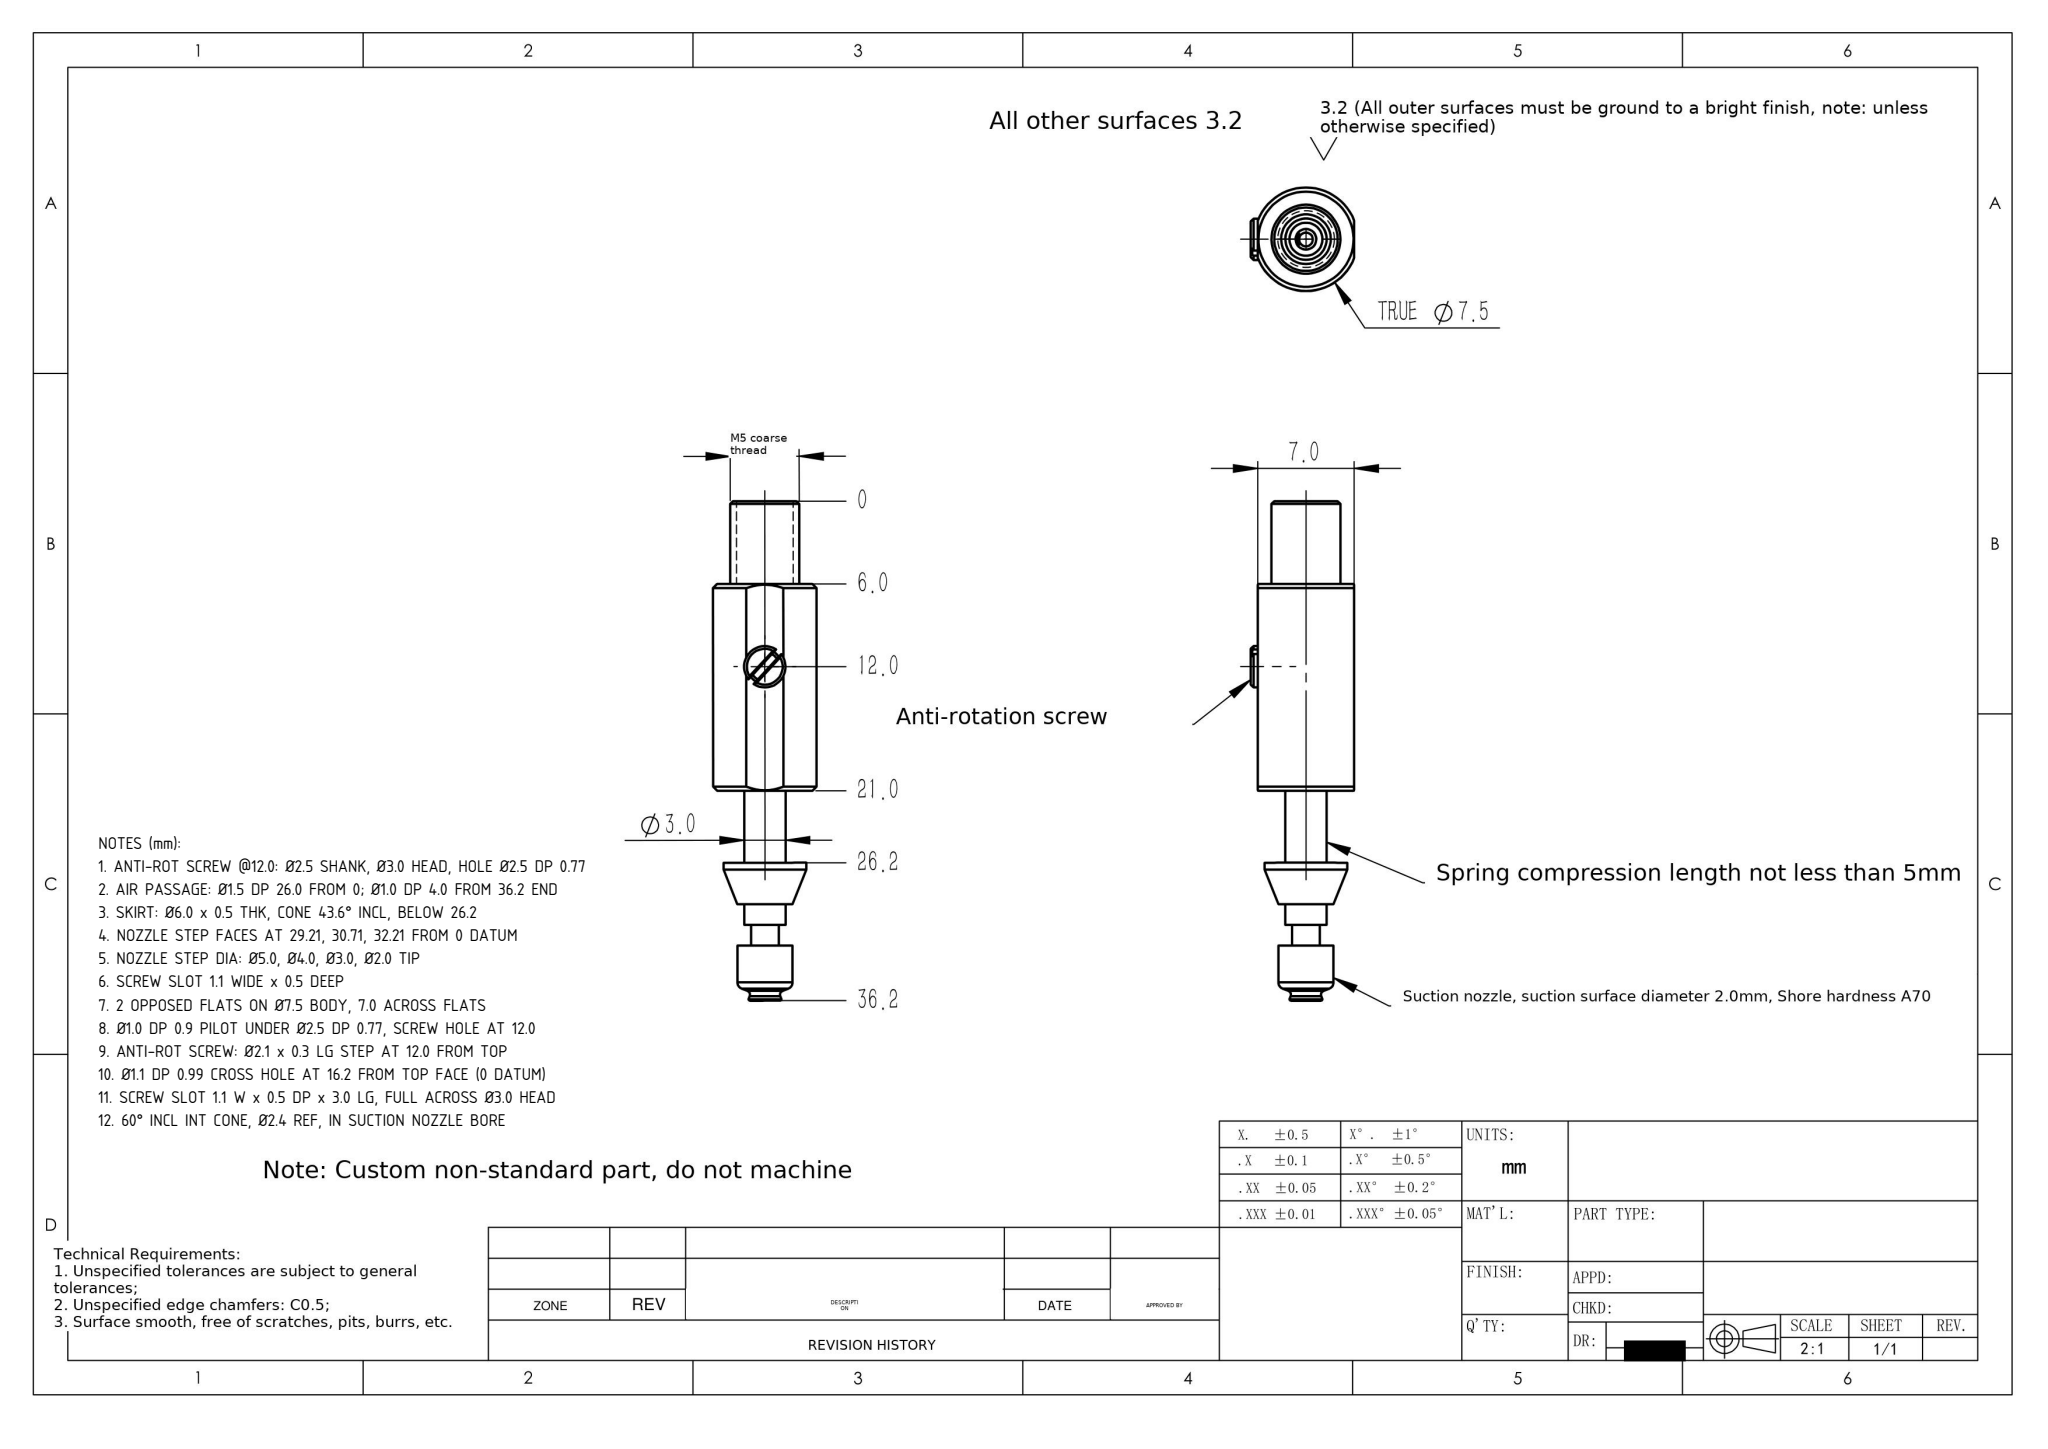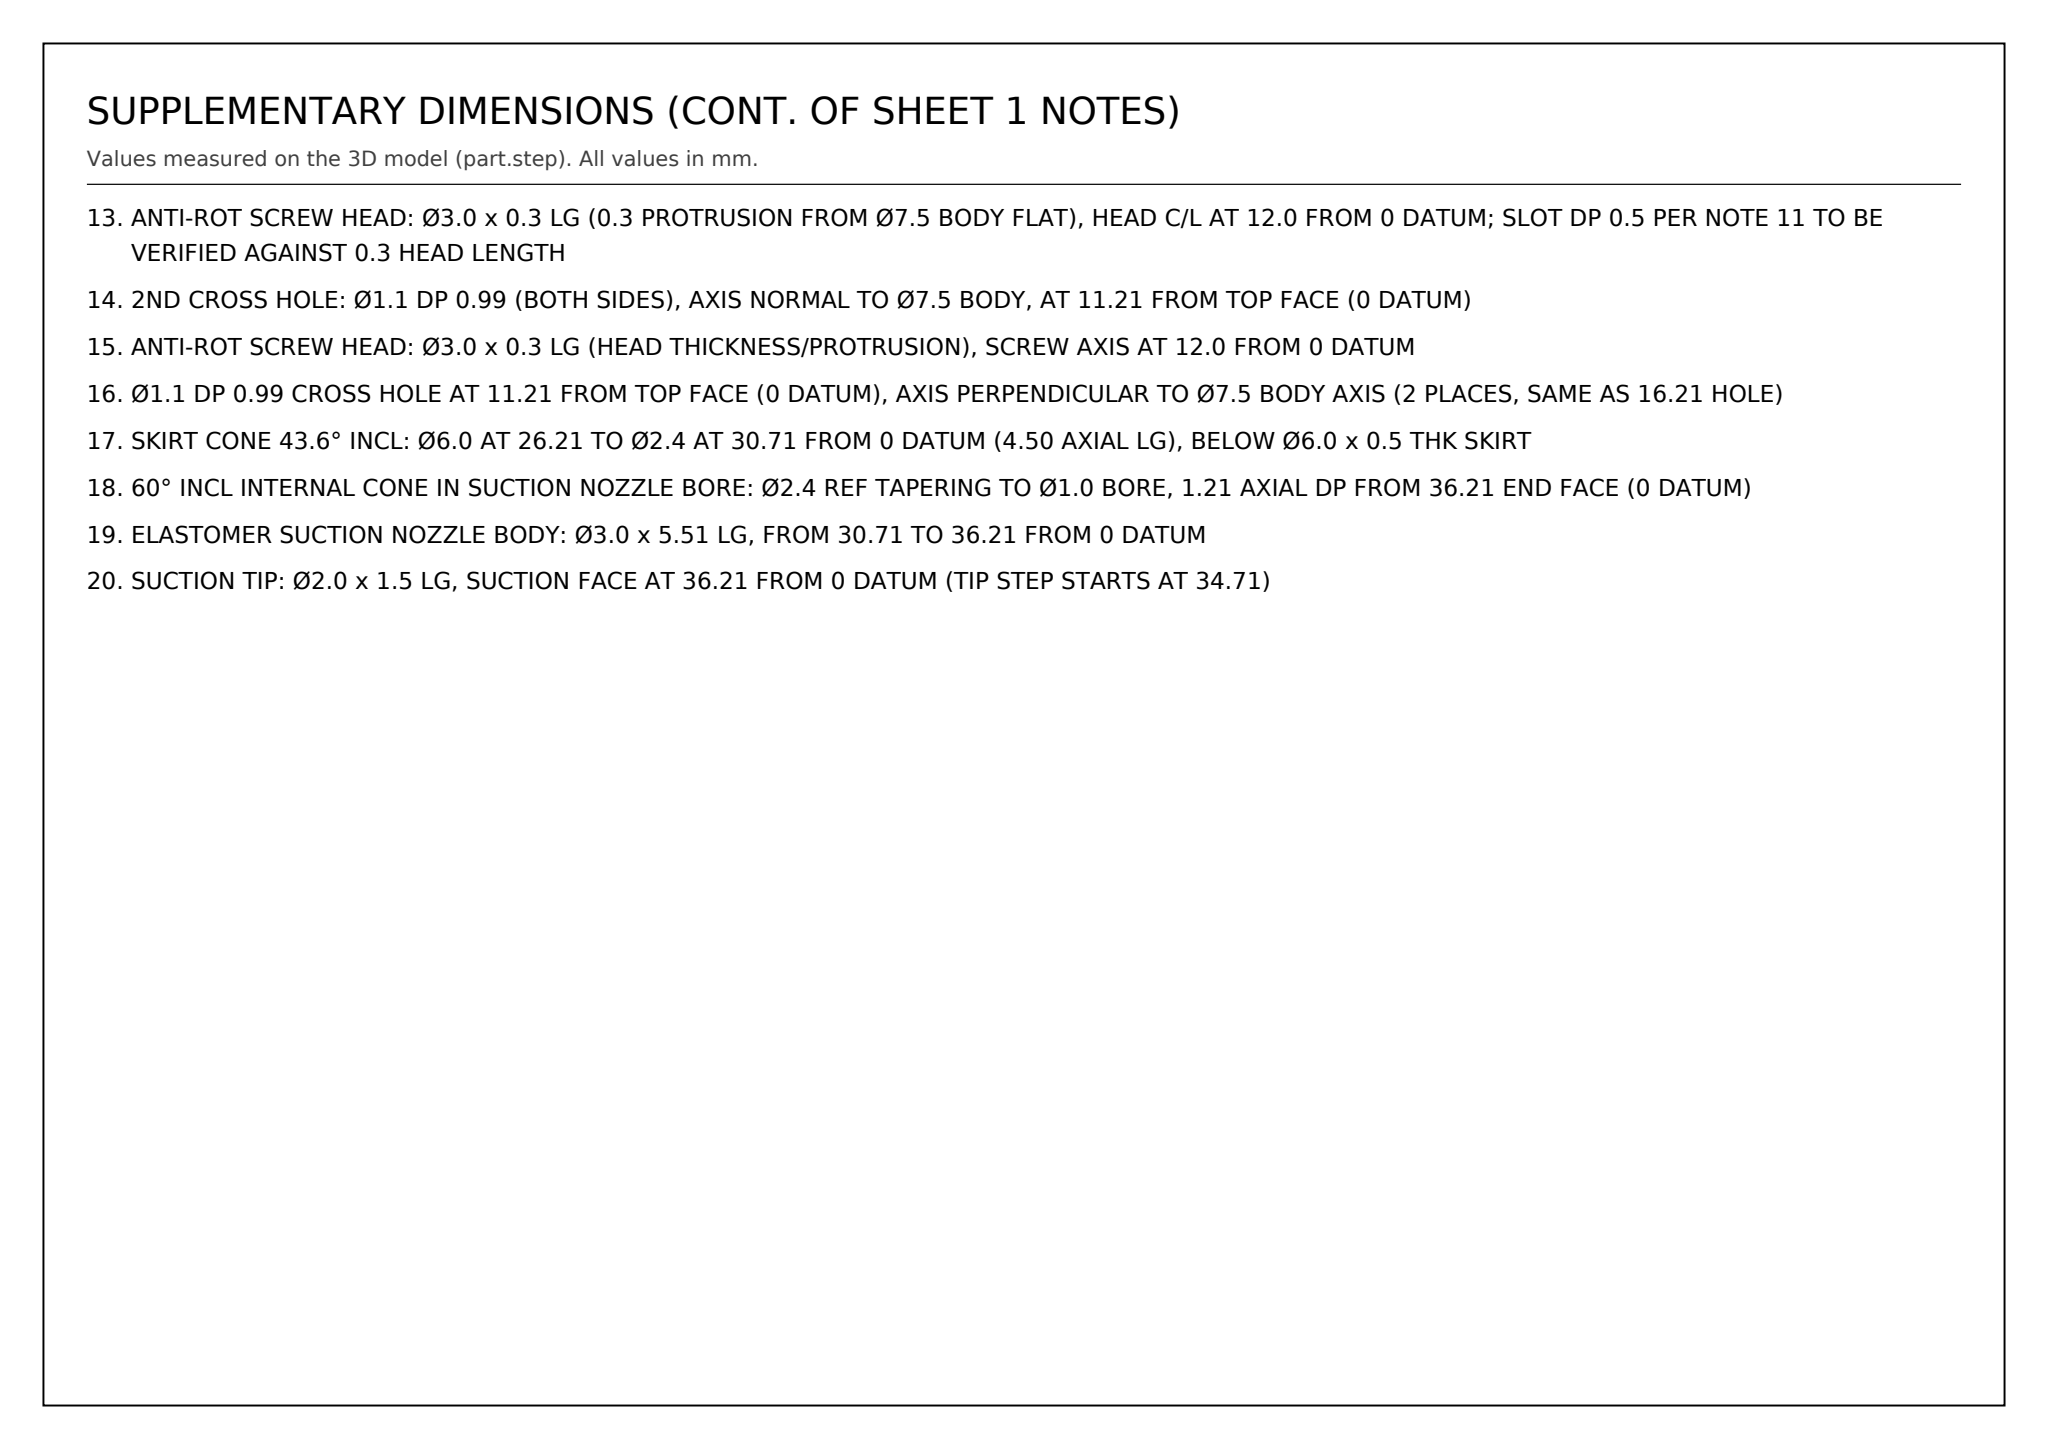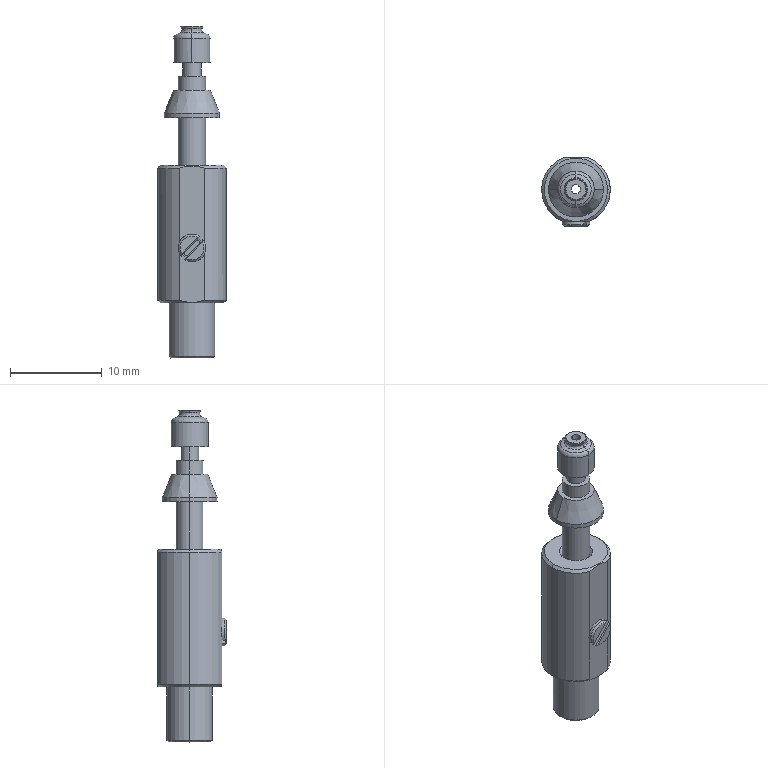Part | SolidWorks | mm | 1 solid | 105 faces | box 7.51 x 7.5 x 36.21 mm | volume 822 mm3 | cylinder 42 | plane 31 | cone 26 | spline 6 | commonest cylinder face diameters 3 x13 1.1 x6 2.5 x4 1 x4 7.5 x3 1.5 x2 6 x2 2 x2
Drawing notes:
ANTI-ROT SCREW @12.0: Ø2.5 SHANK, Ø3.0 HEAD, HOLE Ø2.5 DP 0.77 | from the solid: y-axis cyls at z=12.0: Ø3.0 L0.3, Ø2.5 L0.3 & L0.77, Ø2.1 L0.3, Ø1.0 L0.9
AIR PASSAGE: Ø1.5 DP 26.0 FROM 0; Ø1.0 DP 4.0 FROM 36.2 END | from the solid: z-axis cyls Ø1.5 L26.0 and Ø1.0 L4.0 on axis x4.0 y4.0
SKIRT: Ø6.0 x 0.5 THK, CONE 43.6° INCL, BELOW 26.2 | from the solid: Ø6.0 z-cyl L0.5; cone included angle 43.6° ref dia 6.0; z plane 26.21
NOZZLE STEP FACES AT 29.21, 30.71, 32.21 FROM 0 DATUM | from the solid: z planes 29.21, 30.71, 32.21 between 26.21 and 36.21
NOZZLE STEP DIA: Ø5.0, Ø4.0, Ø3.0, Ø2.0 TIP | from the solid: z-axis cyls Ø5.0 L5.8, Ø4.0 L2.66, Ø3.0 L1.5/2.31, Ø2.0 L1.5
SCREW SLOT 1.1 WIDE x 0.5 DEEP | from the solid: x planes 3.46/4.56 (1.1 apart, ctr x=4.01); y planes 0.0 to 0.5
2 OPPOSED FLATS ON Ø7.5 BODY, 7.0 ACROSS FLATS | from the solid: y planes 0.5 and 7.5 about axis y=4.0 on Ø7.5 L14.4 cyl = 7.0 A/F
Ø1.0 DP 0.9 PILOT UNDER Ø2.5 DP 0.77, SCREW HOLE AT 12.0 | from the solid: cyl Ø1.0 axis Y at (x4.01, z12.0), lg 0.9, below Ø2.5 Y-bore 0.77 dp
ANTI-ROT SCREW: Ø2.1 x 0.3 LG STEP AT 12.0 FROM TOP | from the solid: cyl Ø2.1 axis Y at (x4.01, z12.0), lg 0.3
Ø1.1 DP 0.99 CROSS HOLE AT 16.2 FROM TOP FACE (0 DATUM) | from the solid: cyl Ø1.1 axis Y at (x4.01, z16.21), lg 0.99
SCREW SLOT 1.1 W x 0.5 DP x 3.0 LG, FULL ACROSS Ø3.0 HEAD | from the solid: planes X=3.46 & X=4.56 (1.1 apart); Ø3.0 Y-cyl head at z12.0
60° INCL INT CONE, Ø2.4 REF, IN SUCTION NOZZLE BORE | from the solid: cone included angle 60.0, ref dia 2.4, count 2 (nozzle end of part)
ANTI-ROT SCREW HEAD: Ø3.0 x 0.3 LG (0.3 PROTRUSION FROM Ø7.5 BODY FLAT), HEAD C/L AT 12.0 FROM 0 DATUM; SLOT DP 0.5 PER NOTE 11 TO BE VERIFIED AGAINST 0.3 HEAD LENGTH | from the solid: cylinder [3.0, y-axis, pos (4.01, z=12.0), length 0.3] (screw head), with 2.1 x 0.3 and 2.5 x 0.3 / 2.5 x 0.77 coaxial steps on same y axis
2ND CROSS HOLE: Ø1.1 DP 0.99 (BOTH SIDES), AXIS NORMAL TO Ø7.5 BODY, AT 11.21 FROM TOP FACE (0 DATUM) | from the solid: cylinders [1.1, y-axis, pos (4.01, z=11.21), length 0.99, count 4] distinct from [1.1, y-axis, z=16.21]
ANTI-ROT SCREW HEAD: Ø3.0 x 0.3 LG (HEAD THICKNESS/PROTRUSION), SCREW AXIS AT 12.0 FROM 0 DATUM | from the solid: cylinder [3.0, axis y, pos (4.01, -, 12.0), length 0.3]
Ø1.1 DP 0.99 CROSS HOLE AT 11.21 FROM TOP FACE (0 DATUM), AXIS PERPENDICULAR TO Ø7.5 BODY AXIS (2 PLACES, SAME AS 16.21 HOLE) | from the solid: cylinder [1.1, axis y, pos (4.01, -, 11.21), length 0.99, count 4]
SKIRT CONE 43.6° INCL: Ø6.0 AT 26.21 TO Ø2.4 AT 30.71 FROM 0 DATUM (4.50 AXIAL LG), BELOW Ø6.0 x 0.5 THK SKIRT | from the solid: cones[43.6°, ref_dia 6.0] and cones[43.6°, ref_dia 2.4]; z axis_planes at 26.21 and 30.71; Ø6.0 z-cylinder L0.5
60° INCL INTERNAL CONE IN SUCTION NOZZLE BORE: Ø2.4 REF TAPERING TO Ø1.0 BORE, 1.21 AXIAL DP FROM 36.21 END FACE (0 DATUM) | from the solid: cones[60.0°, ref_dia 2.4]; Ø1.0 z-cylinder L4.0 opening at z=36.21 end face (axial = (2.4-1.0)/2/tan30°)
ELASTOMER SUCTION NOZZLE BODY: Ø3.0 x 5.51 LG, FROM 30.71 TO 36.21 FROM 0 DATUM | from the solid: Ø3.0 z-cylinder L5.51 at x/y 4.02,4.0; z axis_planes 30.71 and 36.21
SUCTION TIP: Ø2.0 x 1.5 LG, SUCTION FACE AT 36.21 FROM 0 DATUM (TIP STEP STARTS AT 34.71) | from the solid: Ø2.0 z-cylinder L1.5 at x/y 4.02,4.0; z axis_plane 36.21